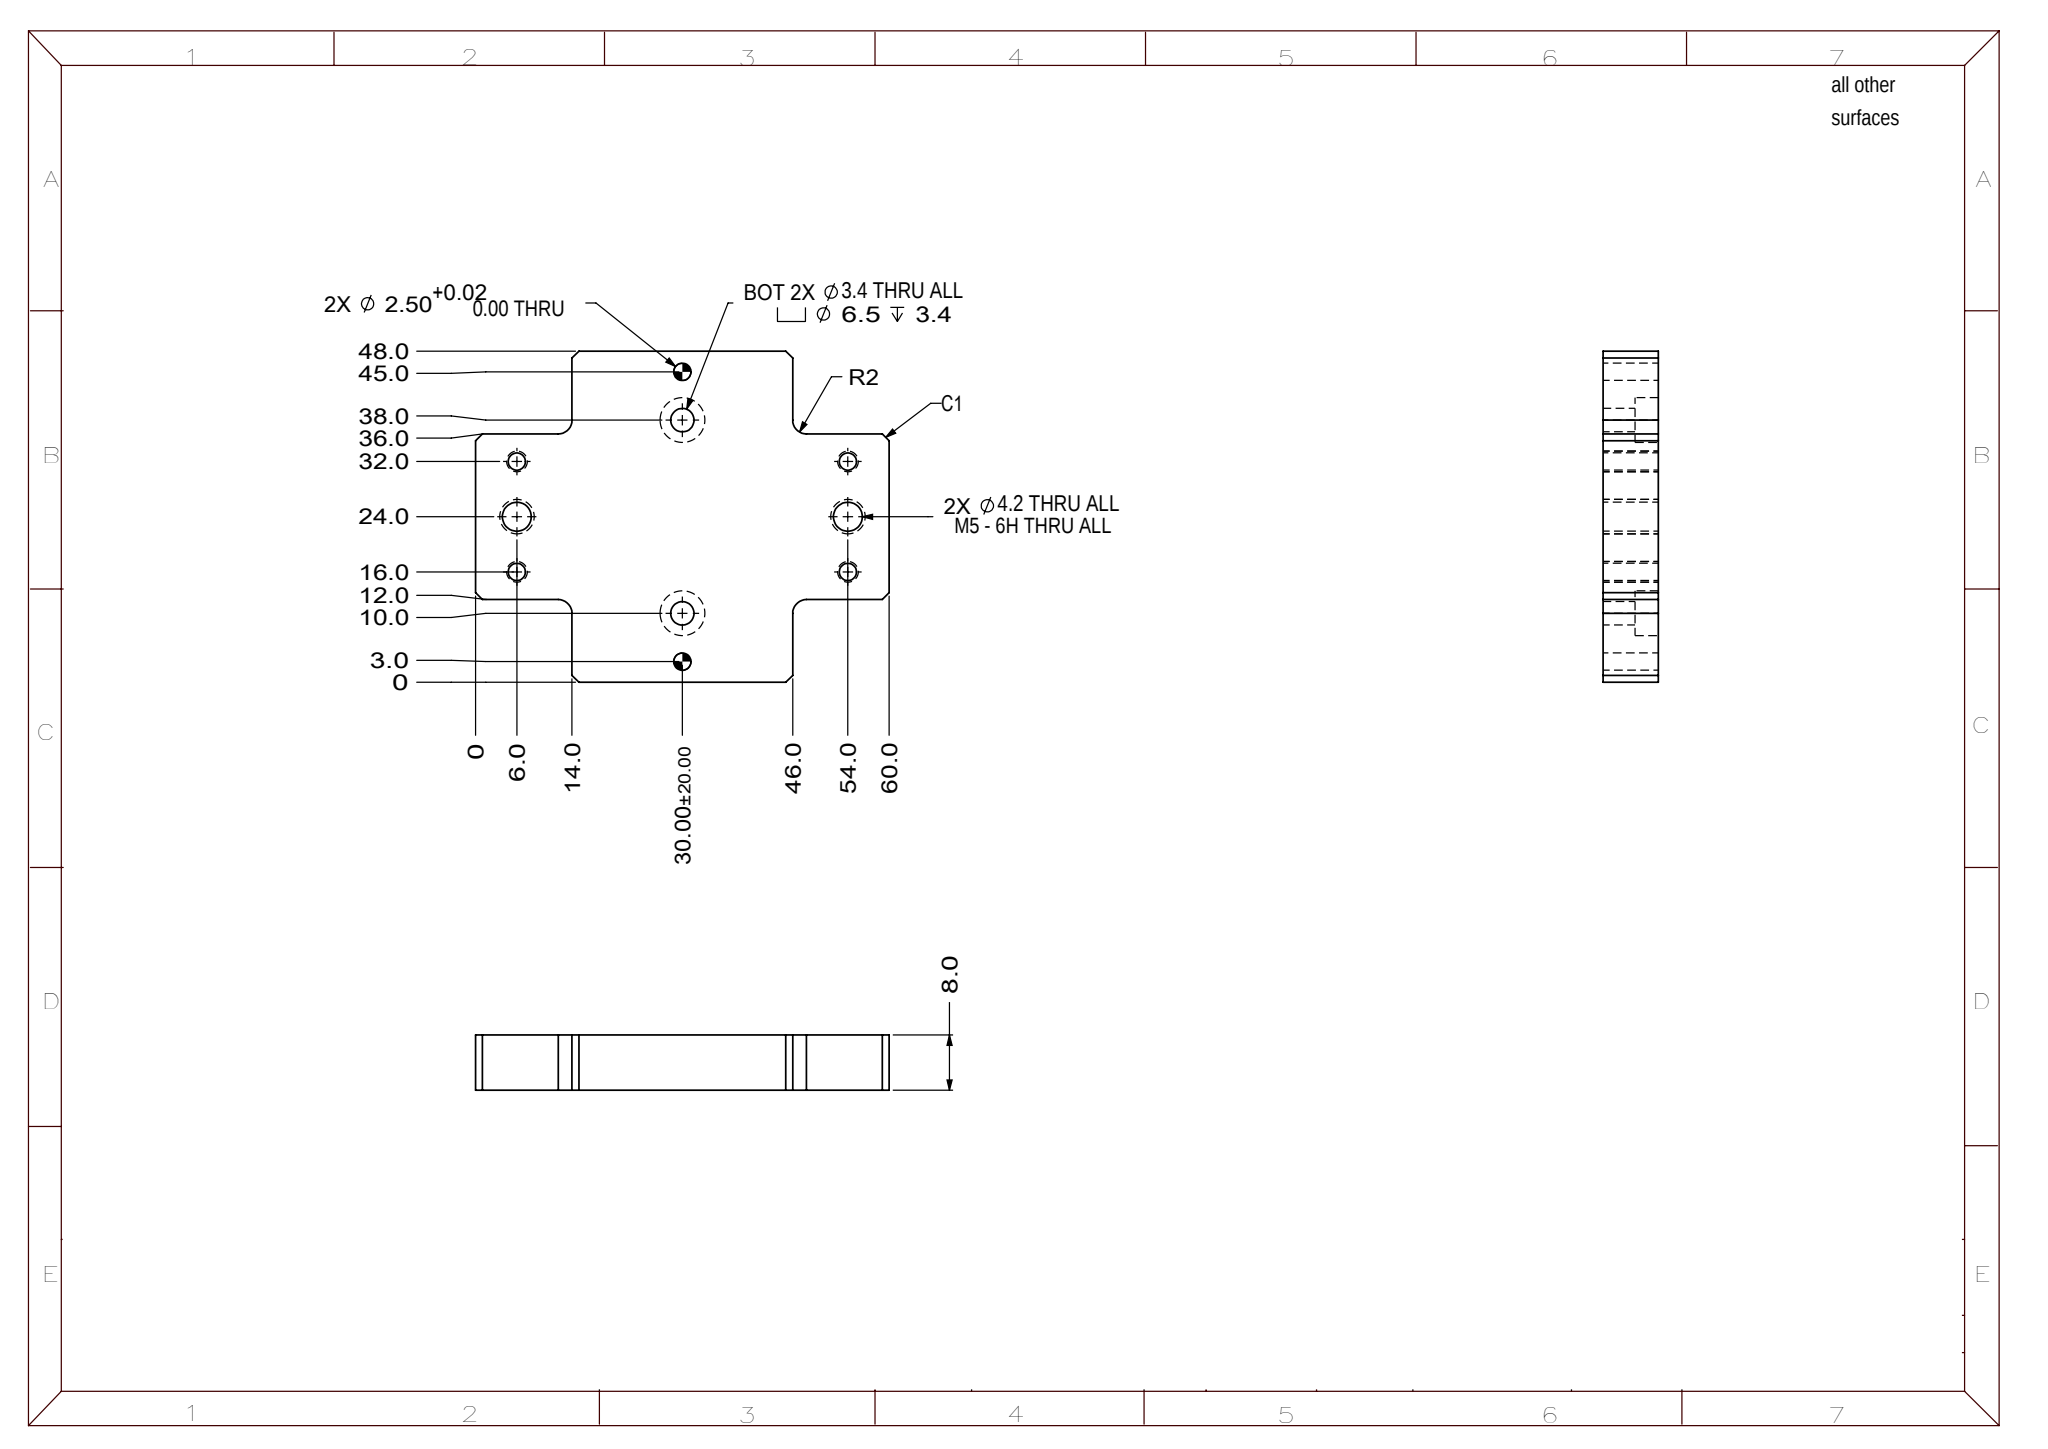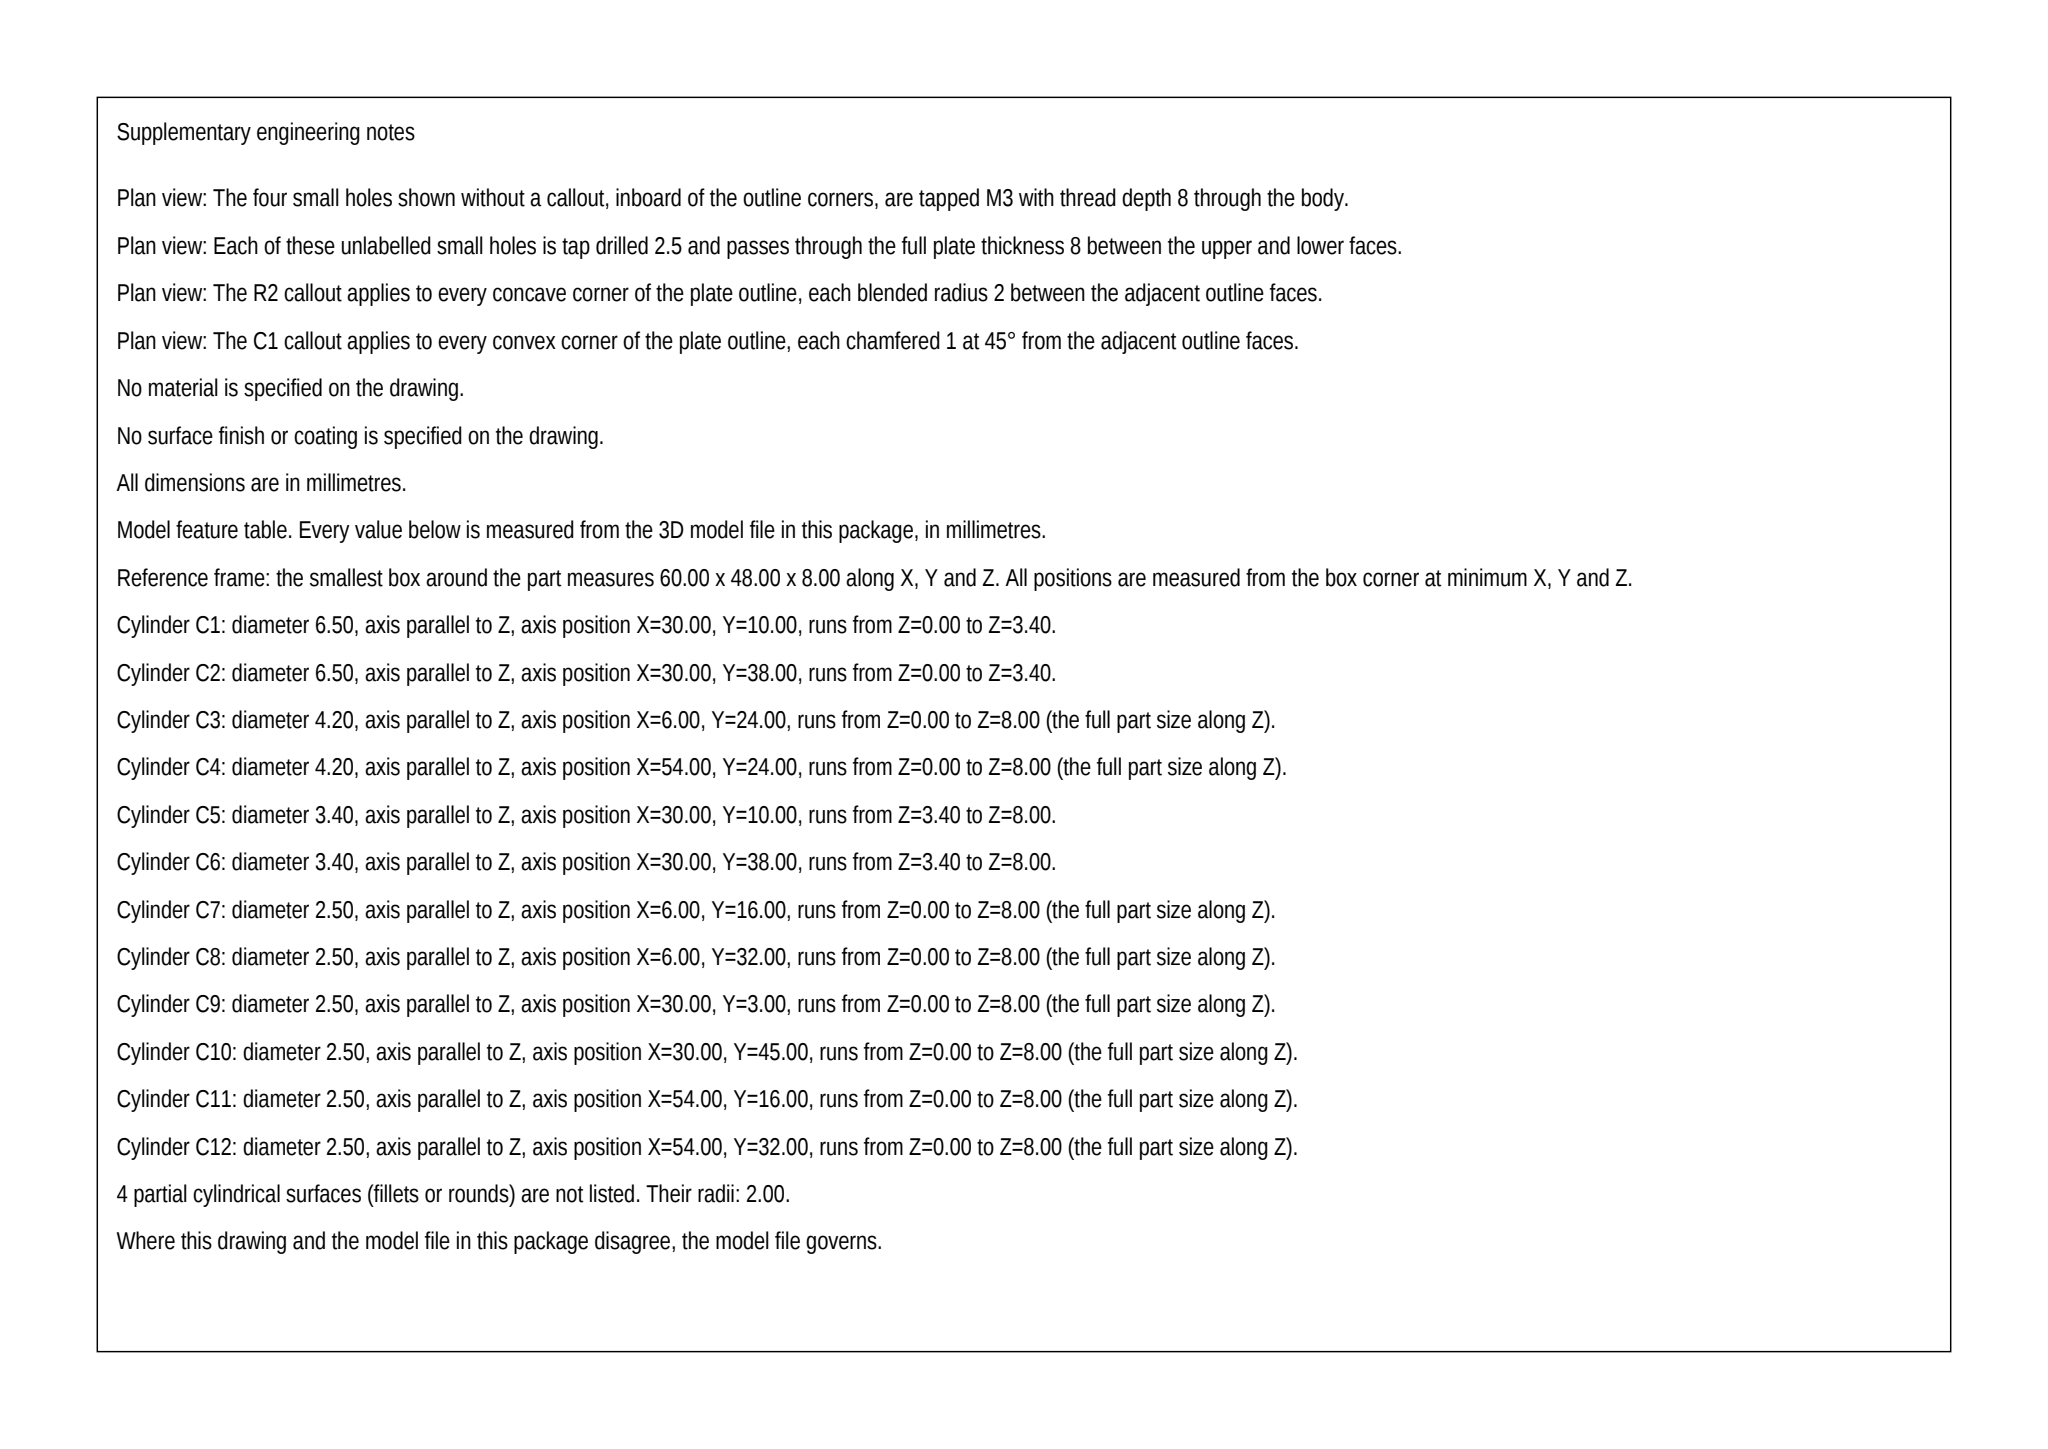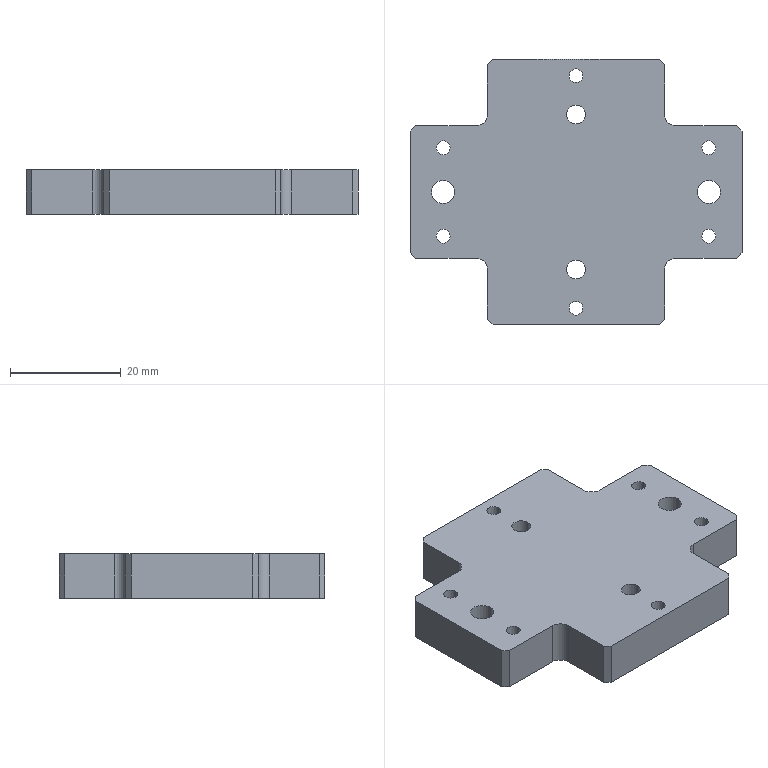Part | SolidWorks | mm | 1 solid | 52 faces | box 60 x 48 x 8 mm | volume 16893 mm3 | cylinder 28 | plane 24 | commonest cylinder face diameters 2.5 x12 6.5 x4 3.4 x4 4.2 x4 4 x4
build123d program:
from build123d import *

# Parameters (mm, degrees)
SKETCH1_W                                       = 60
SKETCH1_H                                       = 48
BOSS_EXTRUDE1_DEPTH                             = 4
SKETCH2_W                                       = 14
SKETCH2_H                                       = 12
CUT_EXTRUDE1_DEPTH                              = 40.243
FILLET1_R                                       = 2
M5_TAPPED_HOLE1_D                               = 4.2
M3_HEX_SOCKET_HEAD_CAP_SCREW_CBORE1_D           = 3.4
M3_HEX_SOCKET_HEAD_CAP_SCREW_CBORE1_CBORE_D     = 6.5
M3_HEX_SOCKET_HEAD_CAP_SCREW_CBORE1_CBORE_DEPTH = 3.4
SIZE_MM_DOWEL_PIN_HOLE1_D                       = 2.5
CHAMFER1_SIZE                                   = 1
M3_TAPPED_HOLE1_D                               = 2.5


with BuildPart() as part:
    # Sketch1 → Boss-Extrude1 (new, symmetric)
    with BuildSketch(Plane.XY):
        Rectangle(SKETCH1_W, SKETCH1_H)
    extrude(amount=BOSS_EXTRUDE1_DEPTH, both=True)

    # Sketch2 → Cut-Extrude1 (cut, through all)
    with BuildSketch(Plane.XY.offset(4)):
        with Locations((-23, 18)):
            Rectangle(SKETCH2_W, SKETCH2_H)
        with Locations((23, 18)):
            Rectangle(SKETCH2_W, SKETCH2_H)
        with Locations((23, -18)):
            Rectangle(SKETCH2_W, SKETCH2_H)
        with Locations((-23, -18)):
            Rectangle(SKETCH2_W, SKETCH2_H)
    extrude(amount=-CUT_EXTRUDE1_DEPTH, mode=Mode.SUBTRACT)

    # Fillet1
    fillet1_edges = [part.edges().sort_by_distance(p)[0] for p in [
        (-16, 12, 0),
        (16, 12, 0),
        (16, -12, 0),
        (-16, -12, 0),
    ]]
    fillet(fillet1_edges, radius=FILLET1_R)

    # M5 Tapped Hole1 (through all)
    with Locations(Plane.XY.offset(4)):
        with Locations((24, 0), (-24, 0)):
            Hole(M5_TAPPED_HOLE1_D / 2)

    # M3 Hex Socket Head Cap Screw CBORE1 (through all)
    with Locations(Plane(origin=(0, 0, -4), x_dir=(-1, 0, 0), z_dir=(0, 0, -1))):
        with Locations((0, 14), (0, -14)):
            CounterBoreHole(M3_HEX_SOCKET_HEAD_CAP_SCREW_CBORE1_D / 2, M3_HEX_SOCKET_HEAD_CAP_SCREW_CBORE1_CBORE_D / 2, M3_HEX_SOCKET_HEAD_CAP_SCREW_CBORE1_CBORE_DEPTH)

    # Size mm Dowel Pin Hole1 (through all)
    with Locations(Plane.XY.offset(4)):
        with Locations((0, 21), (0, -21)):
            Hole(SIZE_MM_DOWEL_PIN_HOLE1_D / 2)

    # Chamfer1
    chamfer1_edges = [part.edges().sort_by_distance(p)[0] for p in [
        (-30, 12, 0),
        (-16, 24, 0),
        (16, 24, 0),
        (30, 12, 0),
        (30, -12, 0),
        (16, -24, 0),
        (-16, -24, 0),
        (-30, -12, 0),
    ]]
    chamfer(chamfer1_edges, length=CHAMFER1_SIZE)

    # M3 Tapped Hole1 (through all)
    with Locations(Plane.XY.offset(4)):
        with Locations((-24, -8), (-24, 8), (24, 8), (24, -8)):
            Hole(M3_TAPPED_HOLE1_D / 2)


solid = part.part